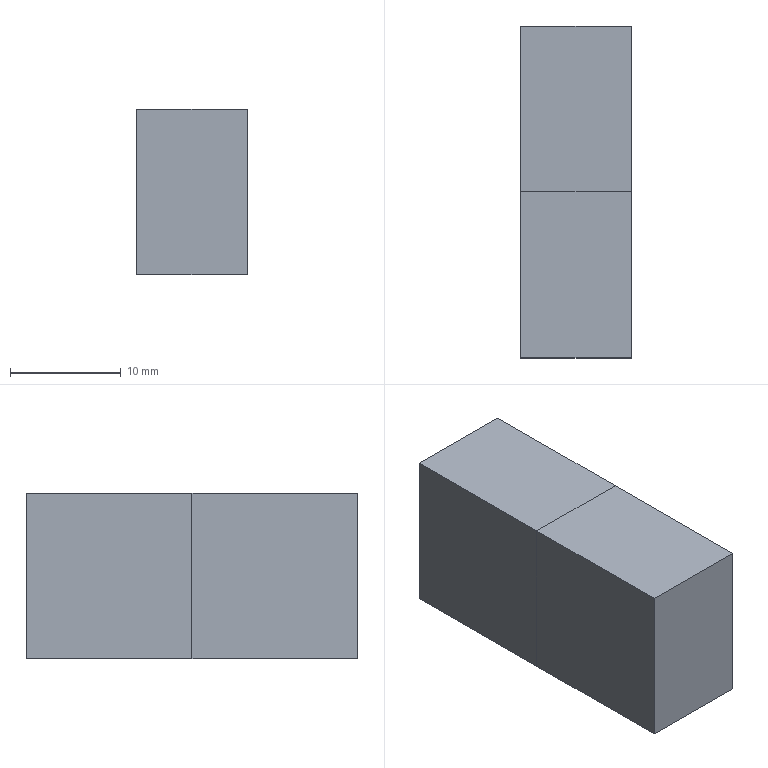Component | NX | 11_OBJECT_2 | 2 solids | 12 faces | box 10 x 30 x 15 mm | volume 4500 mm3 | plane 12
STEP:
#1=CARTESIAN_POINT('',(0.,0.,0.));
#2=DIRECTION('',(0.,0.,1.));
#3=DIRECTION('',(1.,0.,0.));
#4=AXIS2_PLACEMENT_3D('',#1,#2,#3);
#5=CARTESIAN_POINT('',(2050.,95.5,562.5));
#6=VERTEX_POINT('',#5);
#7=CARTESIAN_POINT('',(2050.,110.5,562.5));
#8=VERTEX_POINT('',#7);
#9=CARTESIAN_POINT('',(2050.,95.5,562.5));
#10=DIRECTION('',(0.,1.,0.));
#11=VECTOR('',#10,1.);
#12=LINE('',#9,#11);
#13=CARTESIAN_POINT('',(2060.,95.5,562.5));
#14=DIRECTION('',(0.,0.,1.));
#15=DIRECTION('',(0.,1.,0.));
#16=AXIS2_PLACEMENT_3D('',#13,#14,#15);
#17=PLANE('',#16);
#18=CARTESIAN_POINT('',(0.,10.));
#19=DIRECTION('',(1.,0.));
#20=VECTOR('',#19,1.);
#21=LINE('',#18,#20);
#22=(GEOMETRIC_REPRESENTATION_CONTEXT(2)PARAMETRIC_REPRESENTATION_CONTEXT()REPRESENTATION_CONTEXT('',''));
#23=DEFINITIONAL_REPRESENTATION('',(#21),#22);
#24=PCURVE('',#17,#23);
#25=CARTESIAN_POINT('',(2050.,95.5,562.5));
#26=DIRECTION('',(1.,0.,0.));
#27=DIRECTION('',(0.,1.,0.));
#28=AXIS2_PLACEMENT_3D('',#25,#26,#27);
#29=PLANE('',#28);
#30=CARTESIAN_POINT('',(0.,0.));
#31=DIRECTION('',(1.,0.));
#32=VECTOR('',#31,1.);
#33=LINE('',#30,#32);
#34=(GEOMETRIC_REPRESENTATION_CONTEXT(2)PARAMETRIC_REPRESENTATION_CONTEXT()REPRESENTATION_CONTEXT('',''));
#35=DEFINITIONAL_REPRESENTATION('',(#33),#34);
#36=PCURVE('',#29,#35);
#37=SURFACE_CURVE('',#12,(#24,#36),.PCURVE_S1.);
#38=EDGE_CURVE('',#6,#8,#37,.T.);
#39=ORIENTED_EDGE('',*,*,#38,.T.);
#40=CARTESIAN_POINT('',(2060.,110.5,562.5));
#41=VERTEX_POINT('',#40);
#42=CARTESIAN_POINT('',(2060.,110.5,562.5));
#43=DIRECTION('',(-1.,0.,0.));
#44=VECTOR('',#43,1.);
#45=LINE('',#42,#44);
#46=CARTESIAN_POINT('',(15.,0.));
#47=DIRECTION('',(0.,1.));
#48=VECTOR('',#47,1.);
#49=LINE('',#46,#48);
#50=(GEOMETRIC_REPRESENTATION_CONTEXT(2)PARAMETRIC_REPRESENTATION_CONTEXT()REPRESENTATION_CONTEXT('',''));
#51=DEFINITIONAL_REPRESENTATION('',(#49),#50);
#52=PCURVE('',#17,#51);
#53=CARTESIAN_POINT('',(2060.,110.5,562.5));
#54=DIRECTION('',(0.,-1.,0.));
#55=DIRECTION('',(0.,0.,1.));
#56=AXIS2_PLACEMENT_3D('',#53,#54,#55);
#57=PLANE('',#56);
#58=CARTESIAN_POINT('',(0.,0.));
#59=DIRECTION('',(0.,1.));
#60=VECTOR('',#59,1.);
#61=LINE('',#58,#60);
#62=(GEOMETRIC_REPRESENTATION_CONTEXT(2)PARAMETRIC_REPRESENTATION_CONTEXT()REPRESENTATION_CONTEXT('',''));
#63=DEFINITIONAL_REPRESENTATION('',(#61),#62);
#64=PCURVE('',#57,#63);
#65=SURFACE_CURVE('',#45,(#52,#64),.PCURVE_S1.);
#66=EDGE_CURVE('',#41,#8,#65,.T.);
#67=ORIENTED_EDGE('',*,*,#66,.F.);
#68=CARTESIAN_POINT('',(2060.,95.5,562.5));
#69=VERTEX_POINT('',#68);
#70=CARTESIAN_POINT('',(2060.,95.5,562.5));
#71=DIRECTION('',(0.,1.,0.));
#72=VECTOR('',#71,1.);
#73=LINE('',#70,#72);
#74=CARTESIAN_POINT('',(0.,0.));
#75=DIRECTION('',(1.,0.));
#76=VECTOR('',#75,1.);
#77=LINE('',#74,#76);
#78=(GEOMETRIC_REPRESENTATION_CONTEXT(2)PARAMETRIC_REPRESENTATION_CONTEXT()REPRESENTATION_CONTEXT('',''));
#79=DEFINITIONAL_REPRESENTATION('',(#77),#78);
#80=PCURVE('',#17,#79);
#81=CARTESIAN_POINT('',(2060.,95.5,562.5));
#82=DIRECTION('',(1.,0.,0.));
#83=DIRECTION('',(0.,1.,0.));
#84=AXIS2_PLACEMENT_3D('',#81,#82,#83);
#85=PLANE('',#84);
#86=CARTESIAN_POINT('',(0.,0.));
#87=DIRECTION('',(1.,0.));
#88=VECTOR('',#87,1.);
#89=LINE('',#86,#88);
#90=(GEOMETRIC_REPRESENTATION_CONTEXT(2)PARAMETRIC_REPRESENTATION_CONTEXT()REPRESENTATION_CONTEXT('',''));
#91=DEFINITIONAL_REPRESENTATION('',(#89),#90);
#92=PCURVE('',#85,#91);
#93=SURFACE_CURVE('',#73,(#80,#92),.PCURVE_S1.);
#94=EDGE_CURVE('',#69,#41,#93,.T.);
#95=ORIENTED_EDGE('',*,*,#94,.F.);
#96=CARTESIAN_POINT('',(2060.,95.5,562.5));
#97=DIRECTION('',(-1.,0.,0.));
#98=VECTOR('',#97,1.);
#99=LINE('',#96,#98);
#100=CARTESIAN_POINT('',(0.,0.));
#101=DIRECTION('',(0.,1.));
#102=VECTOR('',#101,1.);
#103=LINE('',#100,#102);
#104=(GEOMETRIC_REPRESENTATION_CONTEXT(2)PARAMETRIC_REPRESENTATION_CONTEXT()REPRESENTATION_CONTEXT('',''));
#105=DEFINITIONAL_REPRESENTATION('',(#103),#104);
#106=PCURVE('',#17,#105);
#107=CARTESIAN_POINT('',(2060.,95.5,577.5));
#108=DIRECTION('',(0.,1.,0.));
#109=DIRECTION('',(0.,0.,-1.));
#110=AXIS2_PLACEMENT_3D('',#107,#108,#109);
#111=PLANE('',#110);
#112=CARTESIAN_POINT('',(15.,0.));
#113=DIRECTION('',(0.,1.));
#114=VECTOR('',#113,1.);
#115=LINE('',#112,#114);
#116=(GEOMETRIC_REPRESENTATION_CONTEXT(2)PARAMETRIC_REPRESENTATION_CONTEXT()REPRESENTATION_CONTEXT('',''));
#117=DEFINITIONAL_REPRESENTATION('',(#115),#116);
#118=PCURVE('',#111,#117);
#119=SURFACE_CURVE('',#99,(#106,#118),.PCURVE_S1.);
#120=EDGE_CURVE('',#69,#6,#119,.T.);
#121=ORIENTED_EDGE('',*,*,#120,.T.);
#122=EDGE_LOOP('',(#39,#67,#95,#121));
#123=FACE_BOUND('',#122,.T.);
#124=ADVANCED_FACE('',(#123),#17,.F.);
#125=CARTESIAN_POINT('',(2050.,110.5,577.5));
#126=VERTEX_POINT('',#125);
#127=CARTESIAN_POINT('',(2050.,110.5,562.5));
#128=DIRECTION('',(0.,0.,1.));
#129=VECTOR('',#128,1.);
#130=LINE('',#127,#129);
#131=CARTESIAN_POINT('',(0.,10.));
#132=DIRECTION('',(1.,0.));
#133=VECTOR('',#132,1.);
#134=LINE('',#131,#133);
#135=(GEOMETRIC_REPRESENTATION_CONTEXT(2)PARAMETRIC_REPRESENTATION_CONTEXT()REPRESENTATION_CONTEXT('',''));
#136=DEFINITIONAL_REPRESENTATION('',(#134),#135);
#137=PCURVE('',#57,#136);
#138=CARTESIAN_POINT('',(15.,0.));
#139=DIRECTION('',(0.,1.));
#140=VECTOR('',#139,1.);
#141=LINE('',#138,#140);
#142=(GEOMETRIC_REPRESENTATION_CONTEXT(2)PARAMETRIC_REPRESENTATION_CONTEXT()REPRESENTATION_CONTEXT('',''));
#143=DEFINITIONAL_REPRESENTATION('',(#141),#142);
#144=PCURVE('',#29,#143);
#145=SURFACE_CURVE('',#130,(#137,#144),.PCURVE_S1.);
#146=EDGE_CURVE('',#8,#126,#145,.T.);
#147=ORIENTED_EDGE('',*,*,#146,.T.);
#148=CARTESIAN_POINT('',(2060.,110.5,577.5));
#149=VERTEX_POINT('',#148);
#150=CARTESIAN_POINT('',(2060.,110.5,577.5));
#151=DIRECTION('',(-1.,0.,0.));
#152=VECTOR('',#151,1.);
#153=LINE('',#150,#152);
#154=CARTESIAN_POINT('',(15.,0.));
#155=DIRECTION('',(0.,1.));
#156=VECTOR('',#155,1.);
#157=LINE('',#154,#156);
#158=(GEOMETRIC_REPRESENTATION_CONTEXT(2)PARAMETRIC_REPRESENTATION_CONTEXT()REPRESENTATION_CONTEXT('',''));
#159=DEFINITIONAL_REPRESENTATION('',(#157),#158);
#160=PCURVE('',#57,#159);
#161=CARTESIAN_POINT('',(2060.,110.5,577.5));
#162=DIRECTION('',(0.,0.,-1.));
#163=DIRECTION('',(0.,-1.,0.));
#164=AXIS2_PLACEMENT_3D('',#161,#162,#163);
#165=PLANE('',#164);
#166=CARTESIAN_POINT('',(0.,0.));
#167=DIRECTION('',(0.,1.));
#168=VECTOR('',#167,1.);
#169=LINE('',#166,#168);
#170=(GEOMETRIC_REPRESENTATION_CONTEXT(2)PARAMETRIC_REPRESENTATION_CONTEXT()REPRESENTATION_CONTEXT('',''));
#171=DEFINITIONAL_REPRESENTATION('',(#169),#170);
#172=PCURVE('',#165,#171);
#173=SURFACE_CURVE('',#153,(#160,#172),.PCURVE_S1.);
#174=EDGE_CURVE('',#149,#126,#173,.T.);
#175=ORIENTED_EDGE('',*,*,#174,.F.);
#176=CARTESIAN_POINT('',(2060.,110.5,562.5));
#177=DIRECTION('',(0.,0.,1.));
#178=VECTOR('',#177,1.);
#179=LINE('',#176,#178);
#180=CARTESIAN_POINT('',(0.,0.));
#181=DIRECTION('',(1.,0.));
#182=VECTOR('',#181,1.);
#183=LINE('',#180,#182);
#184=(GEOMETRIC_REPRESENTATION_CONTEXT(2)PARAMETRIC_REPRESENTATION_CONTEXT()REPRESENTATION_CONTEXT('',''));
#185=DEFINITIONAL_REPRESENTATION('',(#183),#184);
#186=PCURVE('',#57,#185);
#187=CARTESIAN_POINT('',(15.,0.));
#188=DIRECTION('',(0.,1.));
#189=VECTOR('',#188,1.);
#190=LINE('',#187,#189);
#191=(GEOMETRIC_REPRESENTATION_CONTEXT(2)PARAMETRIC_REPRESENTATION_CONTEXT()REPRESENTATION_CONTEXT('',''));
#192=DEFINITIONAL_REPRESENTATION('',(#190),#191);
#193=PCURVE('',#85,#192);
#194=SURFACE_CURVE('',#179,(#186,#193),.PCURVE_S1.);
#195=EDGE_CURVE('',#41,#149,#194,.T.);
#196=ORIENTED_EDGE('',*,*,#195,.F.);
#197=ORIENTED_EDGE('',*,*,#66,.T.);
#198=EDGE_LOOP('',(#147,#175,#196,#197));
#199=FACE_BOUND('',#198,.T.);
#200=ADVANCED_FACE('',(#199),#57,.F.);
#201=CARTESIAN_POINT('',(2050.,95.5,577.5));
#202=VERTEX_POINT('',#201);
#203=CARTESIAN_POINT('',(2050.,110.5,577.5));
#204=DIRECTION('',(0.,-1.,0.));
#205=VECTOR('',#204,1.);
#206=LINE('',#203,#205);
#207=CARTESIAN_POINT('',(0.,10.));
#208=DIRECTION('',(1.,0.));
#209=VECTOR('',#208,1.);
#210=LINE('',#207,#209);
#211=(GEOMETRIC_REPRESENTATION_CONTEXT(2)PARAMETRIC_REPRESENTATION_CONTEXT()REPRESENTATION_CONTEXT('',''));
#212=DEFINITIONAL_REPRESENTATION('',(#210),#211);
#213=PCURVE('',#165,#212);
#214=CARTESIAN_POINT('',(15.,15.));
#215=DIRECTION('',(-1.,0.));
#216=VECTOR('',#215,1.);
#217=LINE('',#214,#216);
#218=(GEOMETRIC_REPRESENTATION_CONTEXT(2)PARAMETRIC_REPRESENTATION_CONTEXT()REPRESENTATION_CONTEXT('',''));
#219=DEFINITIONAL_REPRESENTATION('',(#217),#218);
#220=PCURVE('',#29,#219);
#221=SURFACE_CURVE('',#206,(#213,#220),.PCURVE_S1.);
#222=EDGE_CURVE('',#126,#202,#221,.T.);
#223=ORIENTED_EDGE('',*,*,#222,.T.);
#224=CARTESIAN_POINT('',(2060.,95.5,577.5));
#225=VERTEX_POINT('',#224);
#226=CARTESIAN_POINT('',(2060.,95.5,577.5));
#227=DIRECTION('',(-1.,0.,0.));
#228=VECTOR('',#227,1.);
#229=LINE('',#226,#228);
#230=CARTESIAN_POINT('',(15.,0.));
#231=DIRECTION('',(0.,1.));
#232=VECTOR('',#231,1.);
#233=LINE('',#230,#232);
#234=(GEOMETRIC_REPRESENTATION_CONTEXT(2)PARAMETRIC_REPRESENTATION_CONTEXT()REPRESENTATION_CONTEXT('',''));
#235=DEFINITIONAL_REPRESENTATION('',(#233),#234);
#236=PCURVE('',#165,#235);
#237=CARTESIAN_POINT('',(0.,0.));
#238=DIRECTION('',(0.,1.));
#239=VECTOR('',#238,1.);
#240=LINE('',#237,#239);
#241=(GEOMETRIC_REPRESENTATION_CONTEXT(2)PARAMETRIC_REPRESENTATION_CONTEXT()REPRESENTATION_CONTEXT('',''));
#242=DEFINITIONAL_REPRESENTATION('',(#240),#241);
#243=PCURVE('',#111,#242);
#244=SURFACE_CURVE('',#229,(#236,#243),.PCURVE_S1.);
#245=EDGE_CURVE('',#225,#202,#244,.T.);
#246=ORIENTED_EDGE('',*,*,#245,.F.);
#247=CARTESIAN_POINT('',(2060.,110.5,577.5));
#248=DIRECTION('',(0.,-1.,0.));
#249=VECTOR('',#248,1.);
#250=LINE('',#247,#249);
#251=CARTESIAN_POINT('',(0.,0.));
#252=DIRECTION('',(1.,0.));
#253=VECTOR('',#252,1.);
#254=LINE('',#251,#253);
#255=(GEOMETRIC_REPRESENTATION_CONTEXT(2)PARAMETRIC_REPRESENTATION_CONTEXT()REPRESENTATION_CONTEXT('',''));
#256=DEFINITIONAL_REPRESENTATION('',(#254),#255);
#257=PCURVE('',#165,#256);
#258=CARTESIAN_POINT('',(15.,15.));
#259=DIRECTION('',(-1.,0.));
#260=VECTOR('',#259,1.);
#261=LINE('',#258,#260);
#262=(GEOMETRIC_REPRESENTATION_CONTEXT(2)PARAMETRIC_REPRESENTATION_CONTEXT()REPRESENTATION_CONTEXT('',''));
#263=DEFINITIONAL_REPRESENTATION('',(#261),#262);
#264=PCURVE('',#85,#263);
#265=SURFACE_CURVE('',#250,(#257,#264),.PCURVE_S1.);
#266=EDGE_CURVE('',#149,#225,#265,.T.);
#267=ORIENTED_EDGE('',*,*,#266,.F.);
#268=ORIENTED_EDGE('',*,*,#174,.T.);
#269=EDGE_LOOP('',(#223,#246,#267,#268));
#270=FACE_BOUND('',#269,.T.);
#271=ADVANCED_FACE('',(#270),#165,.F.);
#272=CARTESIAN_POINT('',(2050.,95.5,577.5));
#273=DIRECTION('',(0.,0.,-1.));
#274=VECTOR('',#273,1.);
#275=LINE('',#272,#274);
#276=CARTESIAN_POINT('',(0.,10.));
#277=DIRECTION('',(1.,0.));
#278=VECTOR('',#277,1.);
#279=LINE('',#276,#278);
#280=(GEOMETRIC_REPRESENTATION_CONTEXT(2)PARAMETRIC_REPRESENTATION_CONTEXT()REPRESENTATION_CONTEXT('',''));
#281=DEFINITIONAL_REPRESENTATION('',(#279),#280);
#282=PCURVE('',#111,#281);
#283=CARTESIAN_POINT('',(0.,15.));
#284=DIRECTION('',(0.,-1.));
#285=VECTOR('',#284,1.);
#286=LINE('',#283,#285);
#287=(GEOMETRIC_REPRESENTATION_CONTEXT(2)PARAMETRIC_REPRESENTATION_CONTEXT()REPRESENTATION_CONTEXT('',''));
#288=DEFINITIONAL_REPRESENTATION('',(#286),#287);
#289=PCURVE('',#29,#288);
#290=SURFACE_CURVE('',#275,(#282,#289),.PCURVE_S1.);
#291=EDGE_CURVE('',#202,#6,#290,.T.);
#292=ORIENTED_EDGE('',*,*,#291,.T.);
#293=ORIENTED_EDGE('',*,*,#120,.F.);
#294=CARTESIAN_POINT('',(2060.,95.5,577.5));
#295=DIRECTION('',(0.,0.,-1.));
#296=VECTOR('',#295,1.);
#297=LINE('',#294,#296);
#298=CARTESIAN_POINT('',(0.,0.));
#299=DIRECTION('',(1.,0.));
#300=VECTOR('',#299,1.);
#301=LINE('',#298,#300);
#302=(GEOMETRIC_REPRESENTATION_CONTEXT(2)PARAMETRIC_REPRESENTATION_CONTEXT()REPRESENTATION_CONTEXT('',''));
#303=DEFINITIONAL_REPRESENTATION('',(#301),#302);
#304=PCURVE('',#111,#303);
#305=CARTESIAN_POINT('',(0.,15.));
#306=DIRECTION('',(0.,-1.));
#307=VECTOR('',#306,1.);
#308=LINE('',#305,#307);
#309=(GEOMETRIC_REPRESENTATION_CONTEXT(2)PARAMETRIC_REPRESENTATION_CONTEXT()REPRESENTATION_CONTEXT('',''));
#310=DEFINITIONAL_REPRESENTATION('',(#308),#309);
#311=PCURVE('',#85,#310);
#312=SURFACE_CURVE('',#297,(#304,#311),.PCURVE_S1.);
#313=EDGE_CURVE('',#225,#69,#312,.T.);
#314=ORIENTED_EDGE('',*,*,#313,.F.);
#315=ORIENTED_EDGE('',*,*,#245,.T.);
#316=EDGE_LOOP('',(#292,#293,#314,#315));
#317=FACE_BOUND('',#316,.T.);
#318=ADVANCED_FACE('',(#317),#111,.F.);
#319=ORIENTED_EDGE('',*,*,#94,.T.);
#320=ORIENTED_EDGE('',*,*,#195,.T.);
#321=ORIENTED_EDGE('',*,*,#266,.T.);
#322=ORIENTED_EDGE('',*,*,#313,.T.);
#323=EDGE_LOOP('',(#319,#320,#321,#322));
#324=FACE_BOUND('',#323,.T.);
#325=ADVANCED_FACE('',(#324),#85,.T.);
#326=ORIENTED_EDGE('',*,*,#38,.F.);
#327=ORIENTED_EDGE('',*,*,#291,.F.);
#328=ORIENTED_EDGE('',*,*,#222,.F.);
#329=ORIENTED_EDGE('',*,*,#146,.F.);
#330=EDGE_LOOP('',(#326,#327,#328,#329));
#331=FACE_BOUND('',#330,.T.);
#332=ADVANCED_FACE('',(#331),#29,.F.);
#333=CLOSED_SHELL('',(#124,#200,#271,#318,#325,#332));
#334=MANIFOLD_SOLID_BREP('',#333);
#335=(LENGTH_UNIT()NAMED_UNIT(*)SI_UNIT(.MILLI.,.METRE.));
#336=UNCERTAINTY_MEASURE_WITH_UNIT(LENGTH_MEASURE(0.0000001),#335,'','');
#337=(NAMED_UNIT(*)PLANE_ANGLE_UNIT()SI_UNIT($,.RADIAN.));
#338=(NAMED_UNIT(*)SI_UNIT($,.STERADIAN.)SOLID_ANGLE_UNIT());
#339=(GEOMETRIC_REPRESENTATION_CONTEXT(3)GLOBAL_UNCERTAINTY_ASSIGNED_CONTEXT((#336))GLOBAL_UNIT_ASSIGNED_CONTEXT((#335,#337,#338))REPRESENTATION_CONTEXT('',''));
#340=ADVANCED_BREP_SHAPE_REPRESENTATION('',(#4,#334),#339);
#341=CARTESIAN_POINT('',(0.,0.,0.));
#342=DIRECTION('',(0.,0.,1.));
#343=DIRECTION('',(1.,0.,0.));
#344=AXIS2_PLACEMENT_3D('',#341,#342,#343);
#345=CARTESIAN_POINT('',(0.,0.,0.));
#346=DIRECTION('',(0.,0.,1.));
#347=DIRECTION('',(1.,0.,0.));
#348=AXIS2_PLACEMENT_3D('',#345,#346,#347);
#349=(LENGTH_UNIT()NAMED_UNIT(*)SI_UNIT(.MILLI.,.METRE.));
#350=UNCERTAINTY_MEASURE_WITH_UNIT(LENGTH_MEASURE(0.0000001),#349,'','');
#351=(NAMED_UNIT(*)PLANE_ANGLE_UNIT()SI_UNIT($,.RADIAN.));
#352=(NAMED_UNIT(*)SI_UNIT($,.STERADIAN.)SOLID_ANGLE_UNIT());
#353=(GEOMETRIC_REPRESENTATION_CONTEXT(3)GLOBAL_UNCERTAINTY_ASSIGNED_CONTEXT((#350))GLOBAL_UNIT_ASSIGNED_CONTEXT((#349,#351,#352))REPRESENTATION_CONTEXT('',''));
#354=SHAPE_REPRESENTATION('',(#4,#344,#348),#353);
#355=ITEM_DEFINED_TRANSFORMATION('','',#4,#344);
#356=(REPRESENTATION_RELATIONSHIP('','',#340,#354)REPRESENTATION_RELATIONSHIP_WITH_TRANSFORMATION(#355)SHAPE_REPRESENTATION_RELATIONSHIP());
#357=CARTESIAN_POINT('',(2050.,80.5,562.5));
#358=VERTEX_POINT('',#357);
#359=CARTESIAN_POINT('',(2050.,95.5,562.5));
#360=VERTEX_POINT('',#359);
#361=CARTESIAN_POINT('',(2050.,80.5,562.5));
#362=DIRECTION('',(0.,1.,0.));
#363=VECTOR('',#362,1.);
#364=LINE('',#361,#363);
#365=CARTESIAN_POINT('',(2060.,80.5,562.5));
#366=DIRECTION('',(0.,0.,1.));
#367=DIRECTION('',(0.,1.,0.));
#368=AXIS2_PLACEMENT_3D('',#365,#366,#367);
#369=PLANE('',#368);
#370=CARTESIAN_POINT('',(0.,10.));
#371=DIRECTION('',(1.,0.));
#372=VECTOR('',#371,1.);
#373=LINE('',#370,#372);
#374=(GEOMETRIC_REPRESENTATION_CONTEXT(2)PARAMETRIC_REPRESENTATION_CONTEXT()REPRESENTATION_CONTEXT('',''));
#375=DEFINITIONAL_REPRESENTATION('',(#373),#374);
#376=PCURVE('',#369,#375);
#377=CARTESIAN_POINT('',(2050.,80.5,562.5));
#378=DIRECTION('',(1.,0.,0.));
#379=DIRECTION('',(0.,1.,0.));
#380=AXIS2_PLACEMENT_3D('',#377,#378,#379);
#381=PLANE('',#380);
#382=CARTESIAN_POINT('',(0.,0.));
#383=DIRECTION('',(1.,0.));
#384=VECTOR('',#383,1.);
#385=LINE('',#382,#384);
#386=(GEOMETRIC_REPRESENTATION_CONTEXT(2)PARAMETRIC_REPRESENTATION_CONTEXT()REPRESENTATION_CONTEXT('',''));
#387=DEFINITIONAL_REPRESENTATION('',(#385),#386);
#388=PCURVE('',#381,#387);
#389=SURFACE_CURVE('',#364,(#376,#388),.PCURVE_S1.);
#390=EDGE_CURVE('',#358,#360,#389,.T.);
#391=ORIENTED_EDGE('',*,*,#390,.T.);
#392=CARTESIAN_POINT('',(2060.,95.5,562.5));
#393=VERTEX_POINT('',#392);
#394=CARTESIAN_POINT('',(2060.,95.5,562.5));
#395=DIRECTION('',(-1.,0.,0.));
#396=VECTOR('',#395,1.);
#397=LINE('',#394,#396);
#398=CARTESIAN_POINT('',(15.,0.));
#399=DIRECTION('',(0.,1.));
#400=VECTOR('',#399,1.);
#401=LINE('',#398,#400);
#402=(GEOMETRIC_REPRESENTATION_CONTEXT(2)PARAMETRIC_REPRESENTATION_CONTEXT()REPRESENTATION_CONTEXT('',''));
#403=DEFINITIONAL_REPRESENTATION('',(#401),#402);
#404=PCURVE('',#369,#403);
#405=CARTESIAN_POINT('',(2060.,95.5,562.5));
#406=DIRECTION('',(0.,-1.,0.));
#407=DIRECTION('',(0.,0.,1.));
#408=AXIS2_PLACEMENT_3D('',#405,#406,#407);
#409=PLANE('',#408);
#410=CARTESIAN_POINT('',(0.,0.));
#411=DIRECTION('',(0.,1.));
#412=VECTOR('',#411,1.);
#413=LINE('',#410,#412);
#414=(GEOMETRIC_REPRESENTATION_CONTEXT(2)PARAMETRIC_REPRESENTATION_CONTEXT()REPRESENTATION_CONTEXT('',''));
#415=DEFINITIONAL_REPRESENTATION('',(#413),#414);
#416=PCURVE('',#409,#415);
#417=SURFACE_CURVE('',#397,(#404,#416),.PCURVE_S1.);
#418=EDGE_CURVE('',#393,#360,#417,.T.);
#419=ORIENTED_EDGE('',*,*,#418,.F.);
#420=CARTESIAN_POINT('',(2060.,80.5,562.5));
#421=VERTEX_POINT('',#420);
#422=CARTESIAN_POINT('',(2060.,80.5,562.5));
#423=DIRECTION('',(0.,1.,0.));
#424=VECTOR('',#423,1.);
#425=LINE('',#422,#424);
#426=CARTESIAN_POINT('',(0.,0.));
#427=DIRECTION('',(1.,0.));
#428=VECTOR('',#427,1.);
#429=LINE('',#426,#428);
#430=(GEOMETRIC_REPRESENTATION_CONTEXT(2)PARAMETRIC_REPRESENTATION_CONTEXT()REPRESENTATION_CONTEXT('',''));
#431=DEFINITIONAL_REPRESENTATION('',(#429),#430);
#432=PCURVE('',#369,#431);
#433=CARTESIAN_POINT('',(2060.,80.5,562.5));
#434=DIRECTION('',(1.,0.,0.));
#435=DIRECTION('',(0.,1.,0.));
#436=AXIS2_PLACEMENT_3D('',#433,#434,#435);
#437=PLANE('',#436);
#438=CARTESIAN_POINT('',(0.,0.));
#439=DIRECTION('',(1.,0.));
#440=VECTOR('',#439,1.);
#441=LINE('',#438,#440);
#442=(GEOMETRIC_REPRESENTATION_CONTEXT(2)PARAMETRIC_REPRESENTATION_CONTEXT()REPRESENTATION_CONTEXT('',''));
#443=DEFINITIONAL_REPRESENTATION('',(#441),#442);
#444=PCURVE('',#437,#443);
#445=SURFACE_CURVE('',#425,(#432,#444),.PCURVE_S1.);
#446=EDGE_CURVE('',#421,#393,#445,.T.);
#447=ORIENTED_EDGE('',*,*,#446,.F.);
#448=CARTESIAN_POINT('',(2060.,80.5,562.5));
#449=DIRECTION('',(-1.,0.,0.));
#450=VECTOR('',#449,1.);
#451=LINE('',#448,#450);
#452=CARTESIAN_POINT('',(0.,0.));
#453=DIRECTION('',(0.,1.));
#454=VECTOR('',#453,1.);
#455=LINE('',#452,#454);
#456=(GEOMETRIC_REPRESENTATION_CONTEXT(2)PARAMETRIC_REPRESENTATION_CONTEXT()REPRESENTATION_CONTEXT('',''));
#457=DEFINITIONAL_REPRESENTATION('',(#455),#456);
#458=PCURVE('',#369,#457);
#459=CARTESIAN_POINT('',(2060.,80.5,577.5));
#460=DIRECTION('',(0.,1.,0.));
#461=DIRECTION('',(0.,0.,-1.));
#462=AXIS2_PLACEMENT_3D('',#459,#460,#461);
#463=PLANE('',#462);
#464=CARTESIAN_POINT('',(15.,0.));
#465=DIRECTION('',(0.,1.));
#466=VECTOR('',#465,1.);
#467=LINE('',#464,#466);
#468=(GEOMETRIC_REPRESENTATION_CONTEXT(2)PARAMETRIC_REPRESENTATION_CONTEXT()REPRESENTATION_CONTEXT('',''));
#469=DEFINITIONAL_REPRESENTATION('',(#467),#468);
#470=PCURVE('',#463,#469);
#471=SURFACE_CURVE('',#451,(#458,#470),.PCURVE_S1.);
#472=EDGE_CURVE('',#421,#358,#471,.T.);
#473=ORIENTED_EDGE('',*,*,#472,.T.);
#474=EDGE_LOOP('',(#391,#419,#447,#473));
#475=FACE_BOUND('',#474,.T.);
#476=ADVANCED_FACE('',(#475),#369,.F.);
#477=CARTESIAN_POINT('',(2050.,95.5,577.5));
#478=VERTEX_POINT('',#477);
#479=CARTESIAN_POINT('',(2050.,95.5,562.5));
#480=DIRECTION('',(0.,0.,1.));
#481=VECTOR('',#480,1.);
#482=LINE('',#479,#481);
#483=CARTESIAN_POINT('',(0.,10.));
#484=DIRECTION('',(1.,0.));
#485=VECTOR('',#484,1.);
#486=LINE('',#483,#485);
#487=(GEOMETRIC_REPRESENTATION_CONTEXT(2)PARAMETRIC_REPRESENTATION_CONTEXT()REPRESENTATION_CONTEXT('',''));
#488=DEFINITIONAL_REPRESENTATION('',(#486),#487);
#489=PCURVE('',#409,#488);
#490=CARTESIAN_POINT('',(15.,0.));
#491=DIRECTION('',(0.,1.));
#492=VECTOR('',#491,1.);
#493=LINE('',#490,#492);
#494=(GEOMETRIC_REPRESENTATION_CONTEXT(2)PARAMETRIC_REPRESENTATION_CONTEXT()REPRESENTATION_CONTEXT('',''));
#495=DEFINITIONAL_REPRESENTATION('',(#493),#494);
#496=PCURVE('',#381,#495);
#497=SURFACE_CURVE('',#482,(#489,#496),.PCURVE_S1.);
#498=EDGE_CURVE('',#360,#478,#497,.T.);
#499=ORIENTED_EDGE('',*,*,#498,.T.);
#500=CARTESIAN_POINT('',(2060.,95.5,577.5));
#501=VERTEX_POINT('',#500);
#502=CARTESIAN_POINT('',(2060.,95.5,577.5));
#503=DIRECTION('',(-1.,0.,0.));
#504=VECTOR('',#503,1.);
#505=LINE('',#502,#504);
#506=CARTESIAN_POINT('',(15.,0.));
#507=DIRECTION('',(0.,1.));
#508=VECTOR('',#507,1.);
#509=LINE('',#506,#508);
#510=(GEOMETRIC_REPRESENTATION_CONTEXT(2)PARAMETRIC_REPRESENTATION_CONTEXT()REPRESENTATION_CONTEXT('',''));
#511=DEFINITIONAL_REPRESENTATION('',(#509),#510);
#512=PCURVE('',#409,#511);
#513=CARTESIAN_POINT('',(2060.,95.5,577.5));
#514=DIRECTION('',(0.,0.,-1.));
#515=DIRECTION('',(0.,-1.,0.));
#516=AXIS2_PLACEMENT_3D('',#513,#514,#515);
#517=PLANE('',#516);
#518=CARTESIAN_POINT('',(0.,0.));
#519=DIRECTION('',(0.,1.));
#520=VECTOR('',#519,1.);
#521=LINE('',#518,#520);
#522=(GEOMETRIC_REPRESENTATION_CONTEXT(2)PARAMETRIC_REPRESENTATION_CONTEXT()REPRESENTATION_CONTEXT('',''));
#523=DEFINITIONAL_REPRESENTATION('',(#521),#522);
#524=PCURVE('',#517,#523);
#525=SURFACE_CURVE('',#505,(#512,#524),.PCURVE_S1.);
#526=EDGE_CURVE('',#501,#478,#525,.T.);
#527=ORIENTED_EDGE('',*,*,#526,.F.);
#528=CARTESIAN_POINT('',(2060.,95.5,562.5));
#529=DIRECTION('',(0.,0.,1.));
#530=VECTOR('',#529,1.);
#531=LINE('',#528,#530);
#532=CARTESIAN_POINT('',(0.,0.));
#533=DIRECTION('',(1.,0.));
#534=VECTOR('',#533,1.);
#535=LINE('',#532,#534);
#536=(GEOMETRIC_REPRESENTATION_CONTEXT(2)PARAMETRIC_REPRESENTATION_CONTEXT()REPRESENTATION_CONTEXT('',''));
#537=DEFINITIONAL_REPRESENTATION('',(#535),#536);
#538=PCURVE('',#409,#537);
#539=CARTESIAN_POINT('',(15.,0.));
#540=DIRECTION('',(0.,1.));
#541=VECTOR('',#540,1.);
#542=LINE('',#539,#541);
#543=(GEOMETRIC_REPRESENTATION_CONTEXT(2)PARAMETRIC_REPRESENTATION_CONTEXT()REPRESENTATION_CONTEXT('',''));
#544=DEFINITIONAL_REPRESENTATION('',(#542),#543);
#545=PCURVE('',#437,#544);
#546=SURFACE_CURVE('',#531,(#538,#545),.PCURVE_S1.);
#547=EDGE_CURVE('',#393,#501,#546,.T.);
#548=ORIENTED_EDGE('',*,*,#547,.F.);
#549=ORIENTED_EDGE('',*,*,#418,.T.);
#550=EDGE_LOOP('',(#499,#527,#548,#549));
#551=FACE_BOUND('',#550,.T.);
#552=ADVANCED_FACE('',(#551),#409,.F.);
#553=CARTESIAN_POINT('',(2050.,80.5,577.5));
#554=VERTEX_POINT('',#553);
#555=CARTESIAN_POINT('',(2050.,95.5,577.5));
#556=DIRECTION('',(0.,-1.,0.));
#557=VECTOR('',#556,1.);
#558=LINE('',#555,#557);
#559=CARTESIAN_POINT('',(0.,10.));
#560=DIRECTION('',(1.,0.));
#561=VECTOR('',#560,1.);
#562=LINE('',#559,#561);
#563=(GEOMETRIC_REPRESENTATION_CONTEXT(2)PARAMETRIC_REPRESENTATION_CONTEXT()REPRESENTATION_CONTEXT('',''));
#564=DEFINITIONAL_REPRESENTATION('',(#562),#563);
#565=PCURVE('',#517,#564);
#566=CARTESIAN_POINT('',(15.,15.));
#567=DIRECTION('',(-1.,0.));
#568=VECTOR('',#567,1.);
#569=LINE('',#566,#568);
#570=(GEOMETRIC_REPRESENTATION_CONTEXT(2)PARAMETRIC_REPRESENTATION_CONTEXT()REPRESENTATION_CONTEXT('',''));
#571=DEFINITIONAL_REPRESENTATION('',(#569),#570);
#572=PCURVE('',#381,#571);
#573=SURFACE_CURVE('',#558,(#565,#572),.PCURVE_S1.);
#574=EDGE_CURVE('',#478,#554,#573,.T.);
#575=ORIENTED_EDGE('',*,*,#574,.T.);
#576=CARTESIAN_POINT('',(2060.,80.5,577.5));
#577=VERTEX_POINT('',#576);
#578=CARTESIAN_POINT('',(2060.,80.5,577.5));
#579=DIRECTION('',(-1.,0.,0.));
#580=VECTOR('',#579,1.);
#581=LINE('',#578,#580);
#582=CARTESIAN_POINT('',(15.,0.));
#583=DIRECTION('',(0.,1.));
#584=VECTOR('',#583,1.);
#585=LINE('',#582,#584);
#586=(GEOMETRIC_REPRESENTATION_CONTEXT(2)PARAMETRIC_REPRESENTATION_CONTEXT()REPRESENTATION_CONTEXT('',''));
#587=DEFINITIONAL_REPRESENTATION('',(#585),#586);
#588=PCURVE('',#517,#587);
#589=CARTESIAN_POINT('',(0.,0.));
#590=DIRECTION('',(0.,1.));
#591=VECTOR('',#590,1.);
#592=LINE('',#589,#591);
#593=(GEOMETRIC_REPRESENTATION_CONTEXT(2)PARAMETRIC_REPRESENTATION_CONTEXT()REPRESENTATION_CONTEXT('',''));
#594=DEFINITIONAL_REPRESENTATION('',(#592),#593);
#595=PCURVE('',#463,#594);
#596=SURFACE_CURVE('',#581,(#588,#595),.PCURVE_S1.);
#597=EDGE_CURVE('',#577,#554,#596,.T.);
#598=ORIENTED_EDGE('',*,*,#597,.F.);
#599=CARTESIAN_POINT('',(2060.,95.5,577.5));
#600=DIRECTION('',(0.,-1.,0.));
#601=VECTOR('',#600,1.);
#602=LINE('',#599,#601);
#603=CARTESIAN_POINT('',(0.,0.));
#604=DIRECTION('',(1.,0.));
#605=VECTOR('',#604,1.);
#606=LINE('',#603,#605);
#607=(GEOMETRIC_REPRESENTATION_CONTEXT(2)PARAMETRIC_REPRESENTATION_CONTEXT()REPRESENTATION_CONTEXT('',''));
#608=DEFINITIONAL_REPRESENTATION('',(#606),#607);
#609=PCURVE('',#517,#608);
#610=CARTESIAN_POINT('',(15.,15.));
#611=DIRECTION('',(-1.,0.));
#612=VECTOR('',#611,1.);
#613=LINE('',#610,#612);
#614=(GEOMETRIC_REPRESENTATION_CONTEXT(2)PARAMETRIC_REPRESENTATION_CONTEXT()REPRESENTATION_CONTEXT('',''));
#615=DEFINITIONAL_REPRESENTATION('',(#613),#614);
#616=PCURVE('',#437,#615);
#617=SURFACE_CURVE('',#602,(#609,#616),.PCURVE_S1.);
#618=EDGE_CURVE('',#501,#577,#617,.T.);
#619=ORIENTED_EDGE('',*,*,#618,.F.);
#620=ORIENTED_EDGE('',*,*,#526,.T.);
#621=EDGE_LOOP('',(#575,#598,#619,#620));
#622=FACE_BOUND('',#621,.T.);
#623=ADVANCED_FACE('',(#622),#517,.F.);
#624=CARTESIAN_POINT('',(2050.,80.5,577.5));
#625=DIRECTION('',(0.,0.,-1.));
#626=VECTOR('',#625,1.);
#627=LINE('',#624,#626);
#628=CARTESIAN_POINT('',(0.,10.));
#629=DIRECTION('',(1.,0.));
#630=VECTOR('',#629,1.);
#631=LINE('',#628,#630);
#632=(GEOMETRIC_REPRESENTATION_CONTEXT(2)PARAMETRIC_REPRESENTATION_CONTEXT()REPRESENTATION_CONTEXT('',''));
#633=DEFINITIONAL_REPRESENTATION('',(#631),#632);
#634=PCURVE('',#463,#633);
#635=CARTESIAN_POINT('',(0.,15.));
#636=DIRECTION('',(0.,-1.));
#637=VECTOR('',#636,1.);
#638=LINE('',#635,#637);
#639=(GEOMETRIC_REPRESENTATION_CONTEXT(2)PARAMETRIC_REPRESENTATION_CONTEXT()REPRESENTATION_CONTEXT('',''));
#640=DEFINITIONAL_REPRESENTATION('',(#638),#639);
#641=PCURVE('',#381,#640);
#642=SURFACE_CURVE('',#627,(#634,#641),.PCURVE_S1.);
#643=EDGE_CURVE('',#554,#358,#642,.T.);
#644=ORIENTED_EDGE('',*,*,#643,.T.);
#645=ORIENTED_EDGE('',*,*,#472,.F.);
#646=CARTESIAN_POINT('',(2060.,80.5,577.5));
#647=DIRECTION('',(0.,0.,-1.));
#648=VECTOR('',#647,1.);
#649=LINE('',#646,#648);
#650=CARTESIAN_POINT('',(0.,0.));
#651=DIRECTION('',(1.,0.));
#652=VECTOR('',#651,1.);
#653=LINE('',#650,#652);
#654=(GEOMETRIC_REPRESENTATION_CONTEXT(2)PARAMETRIC_REPRESENTATION_CONTEXT()REPRESENTATION_CONTEXT('',''));
#655=DEFINITIONAL_REPRESENTATION('',(#653),#654);
#656=PCURVE('',#463,#655);
#657=CARTESIAN_POINT('',(0.,15.));
#658=DIRECTION('',(0.,-1.));
#659=VECTOR('',#658,1.);
#660=LINE('',#657,#659);
#661=(GEOMETRIC_REPRESENTATION_CONTEXT(2)PARAMETRIC_REPRESENTATION_CONTEXT()REPRESENTATION_CONTEXT('',''));
#662=DEFINITIONAL_REPRESENTATION('',(#660),#661);
#663=PCURVE('',#437,#662);
#664=SURFACE_CURVE('',#649,(#656,#663),.PCURVE_S1.);
#665=EDGE_CURVE('',#577,#421,#664,.T.);
#666=ORIENTED_EDGE('',*,*,#665,.F.);
#667=ORIENTED_EDGE('',*,*,#597,.T.);
#668=EDGE_LOOP('',(#644,#645,#666,#667));
#669=FACE_BOUND('',#668,.T.);
#670=ADVANCED_FACE('',(#669),#463,.F.);
#671=ORIENTED_EDGE('',*,*,#446,.T.);
#672=ORIENTED_EDGE('',*,*,#547,.T.);
#673=ORIENTED_EDGE('',*,*,#618,.T.);
#674=ORIENTED_EDGE('',*,*,#665,.T.);
#675=EDGE_LOOP('',(#671,#672,#673,#674));
#676=FACE_BOUND('',#675,.T.);
#677=ADVANCED_FACE('',(#676),#437,.T.);
#678=ORIENTED_EDGE('',*,*,#390,.F.);
#679=ORIENTED_EDGE('',*,*,#643,.F.);
#680=ORIENTED_EDGE('',*,*,#574,.F.);
#681=ORIENTED_EDGE('',*,*,#498,.F.);
#682=EDGE_LOOP('',(#678,#679,#680,#681));
#683=FACE_BOUND('',#682,.T.);
#684=ADVANCED_FACE('',(#683),#381,.F.);
#685=CLOSED_SHELL('',(#476,#552,#623,#670,#677,#684));
#686=MANIFOLD_SOLID_BREP('',#685);
#687=(LENGTH_UNIT()NAMED_UNIT(*)SI_UNIT(.MILLI.,.METRE.));
#688=UNCERTAINTY_MEASURE_WITH_UNIT(LENGTH_MEASURE(0.0000001),#687,'','');
#689=(NAMED_UNIT(*)PLANE_ANGLE_UNIT()SI_UNIT($,.RADIAN.));
#690=(NAMED_UNIT(*)SI_UNIT($,.STERADIAN.)SOLID_ANGLE_UNIT());
#691=(GEOMETRIC_REPRESENTATION_CONTEXT(3)GLOBAL_UNCERTAINTY_ASSIGNED_CONTEXT((#688))GLOBAL_UNIT_ASSIGNED_CONTEXT((#687,#689,#690))REPRESENTATION_CONTEXT('',''));
#692=ADVANCED_BREP_SHAPE_REPRESENTATION('',(#4,#686),#691);
#693=ITEM_DEFINED_TRANSFORMATION('','',#4,#348);
#694=(REPRESENTATION_RELATIONSHIP('','',#692,#354)REPRESENTATION_RELATIONSHIP_WITH_TRANSFORMATION(#693)SHAPE_REPRESENTATION_RELATIONSHIP());